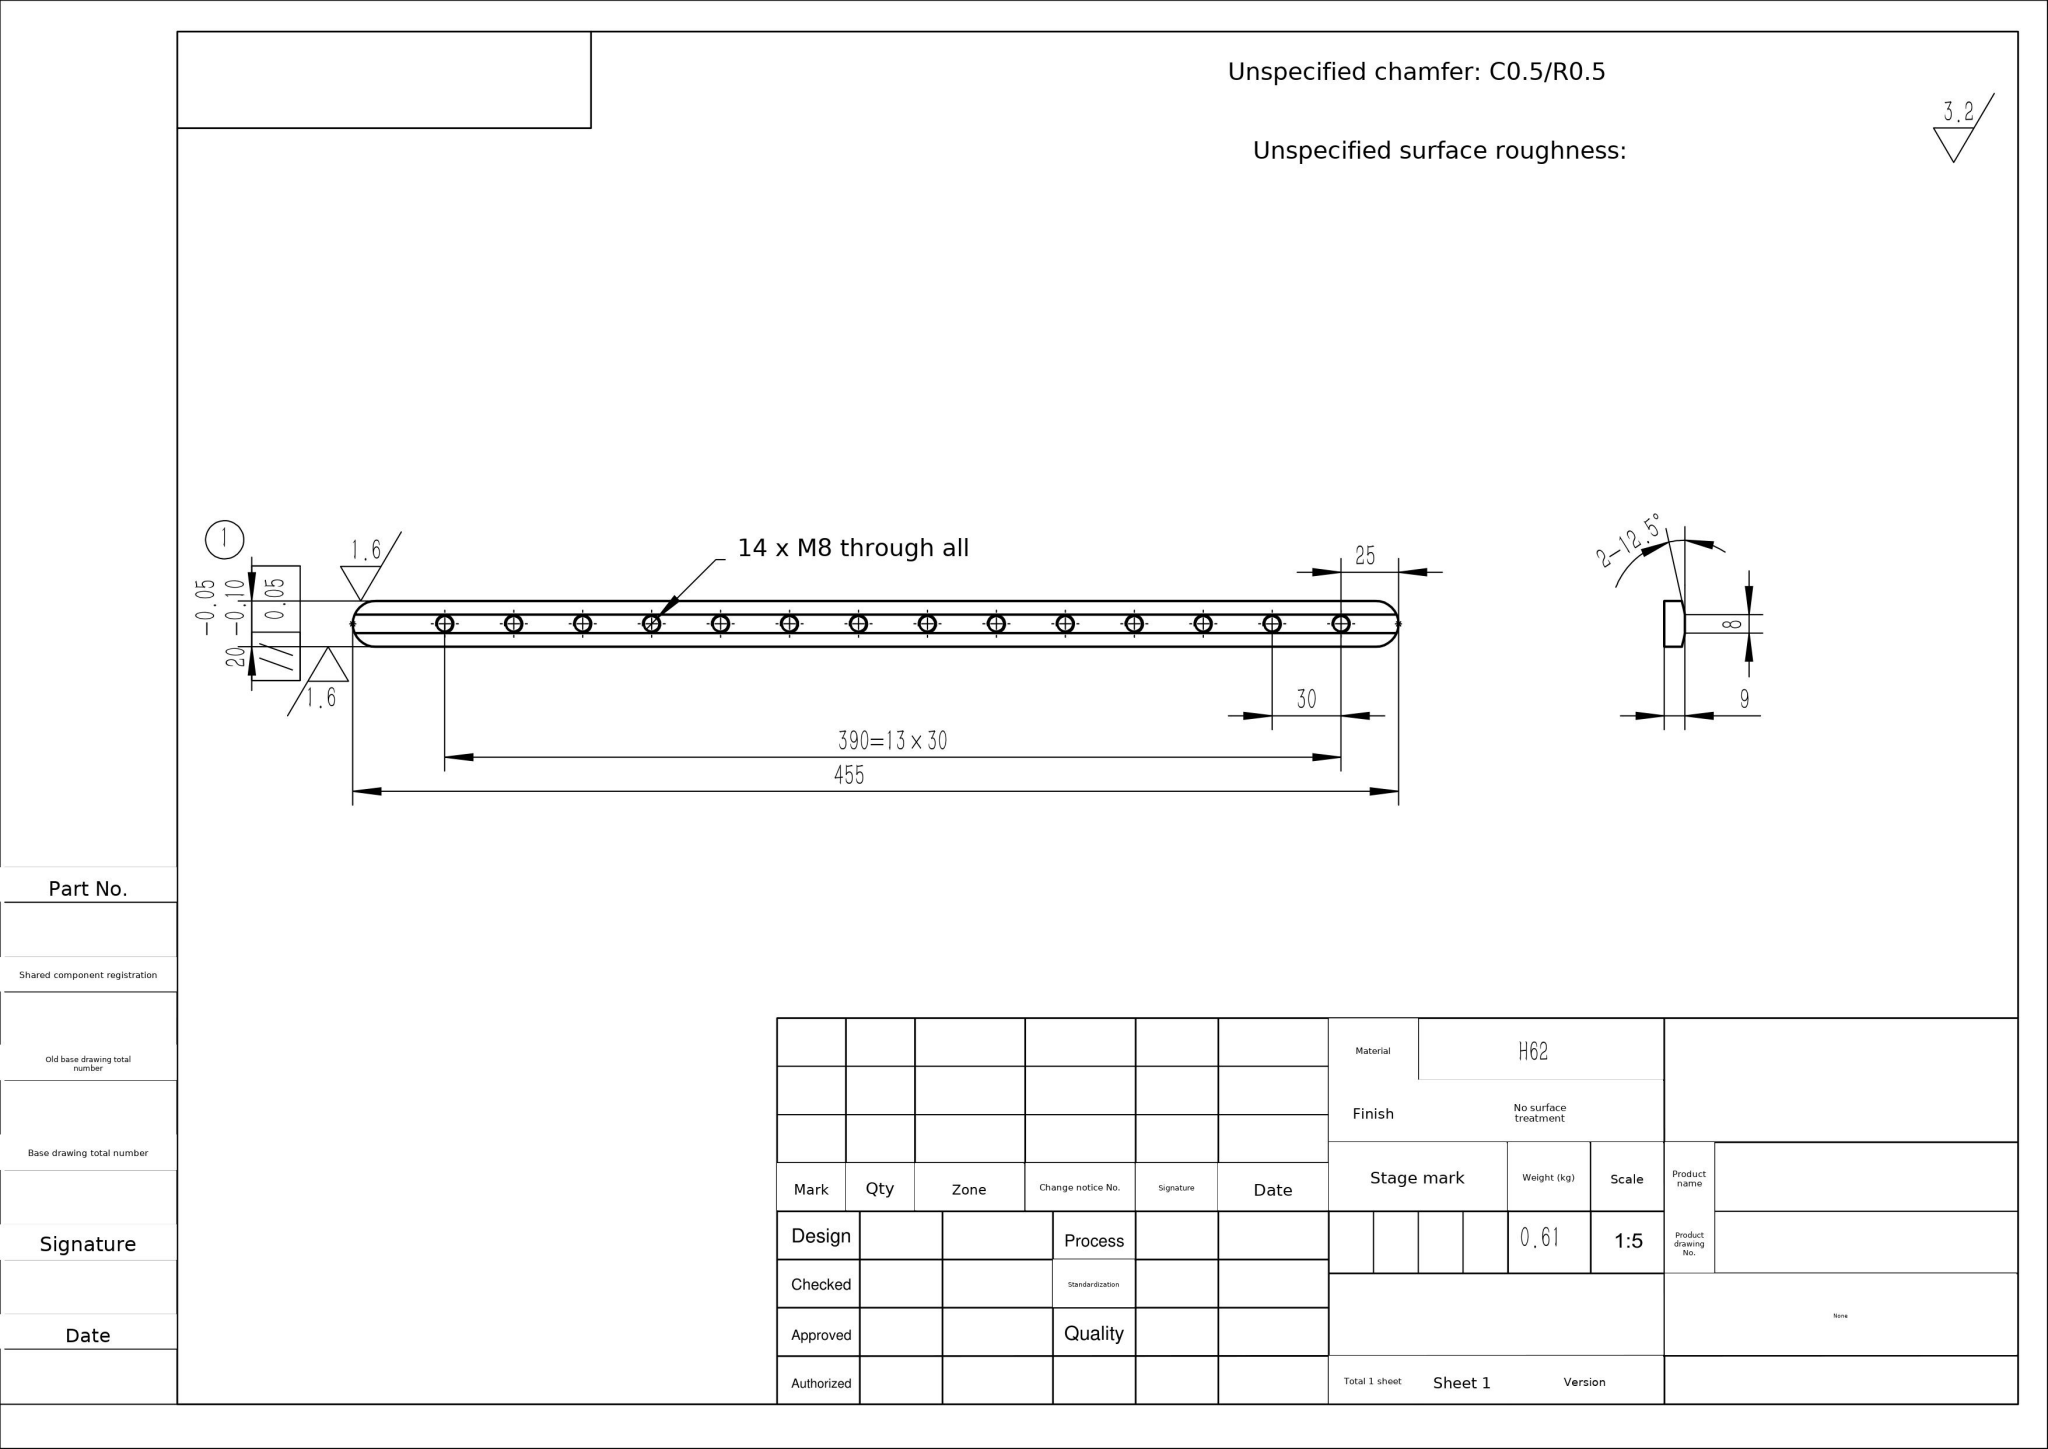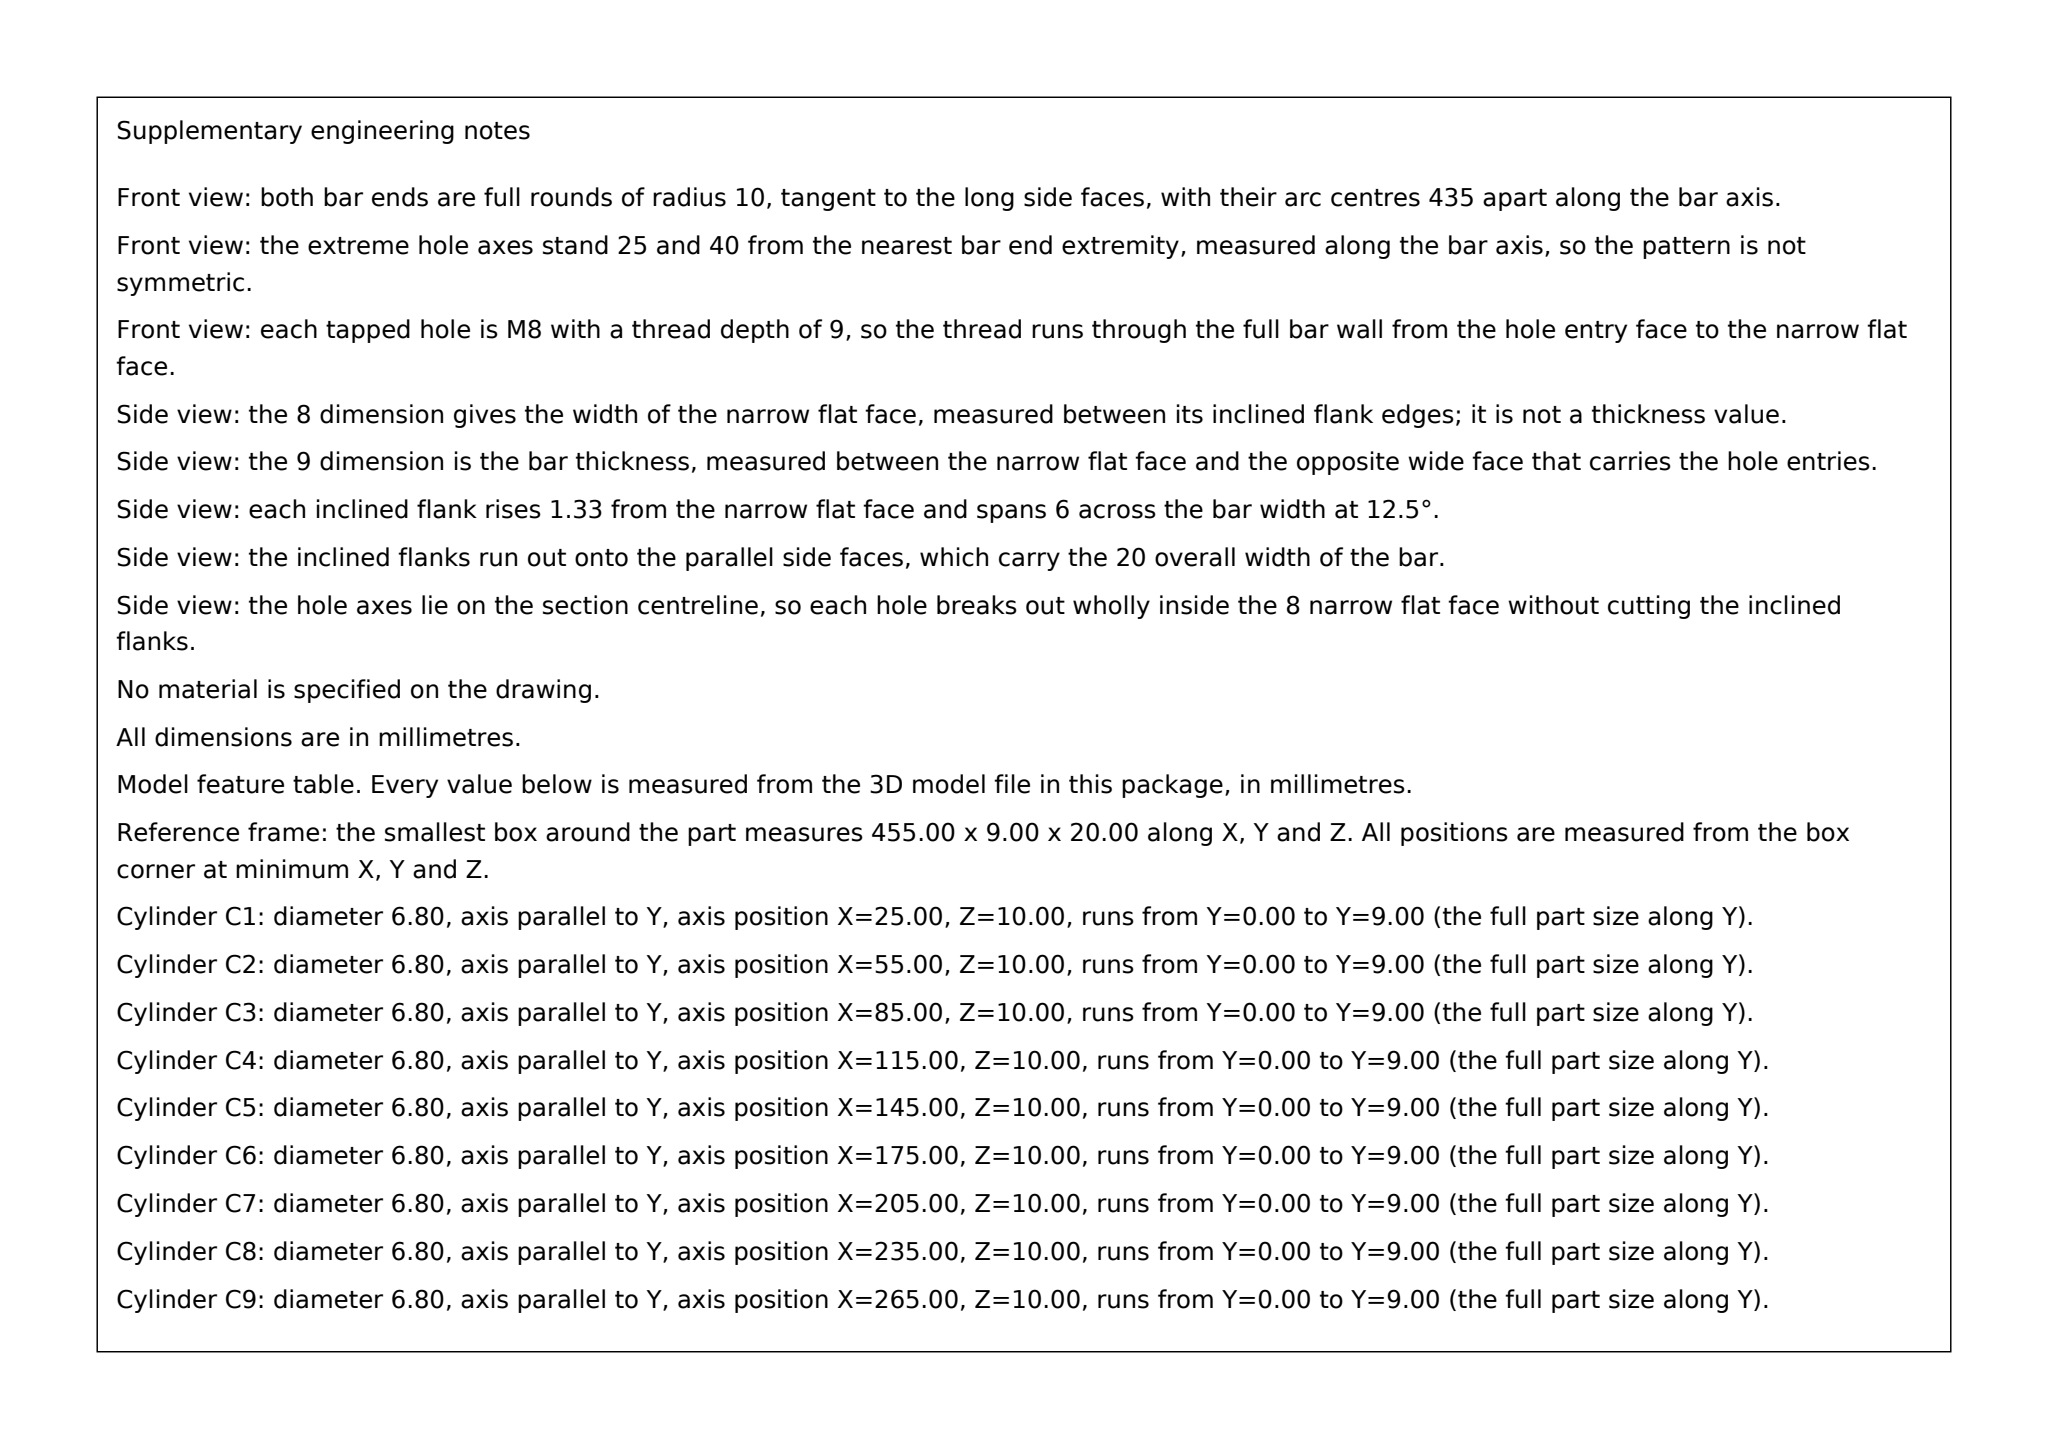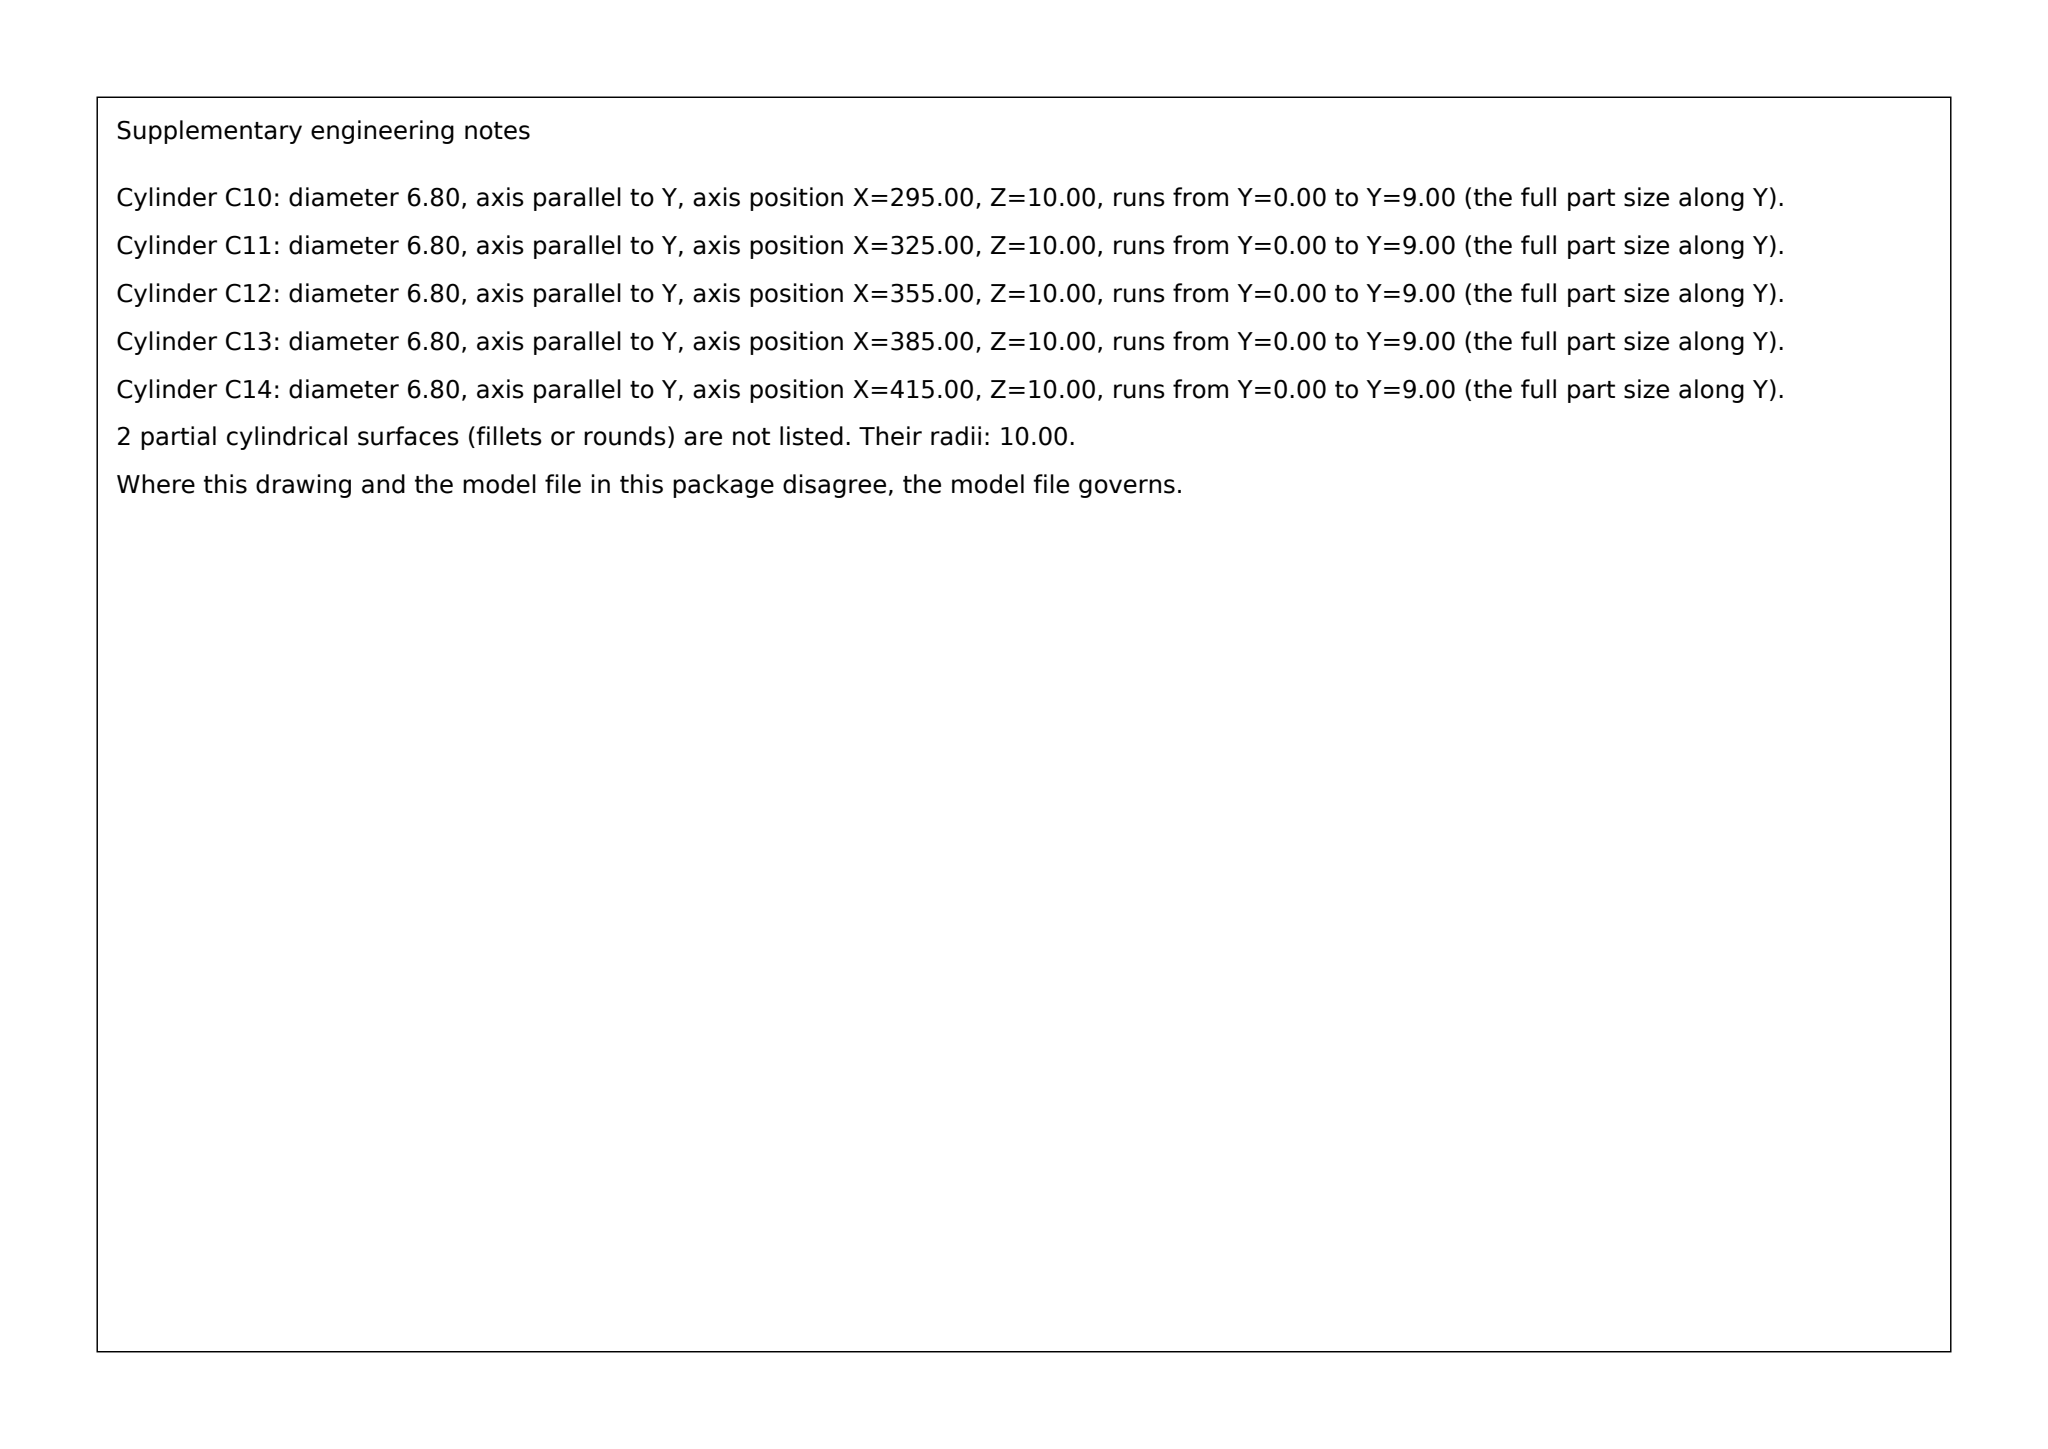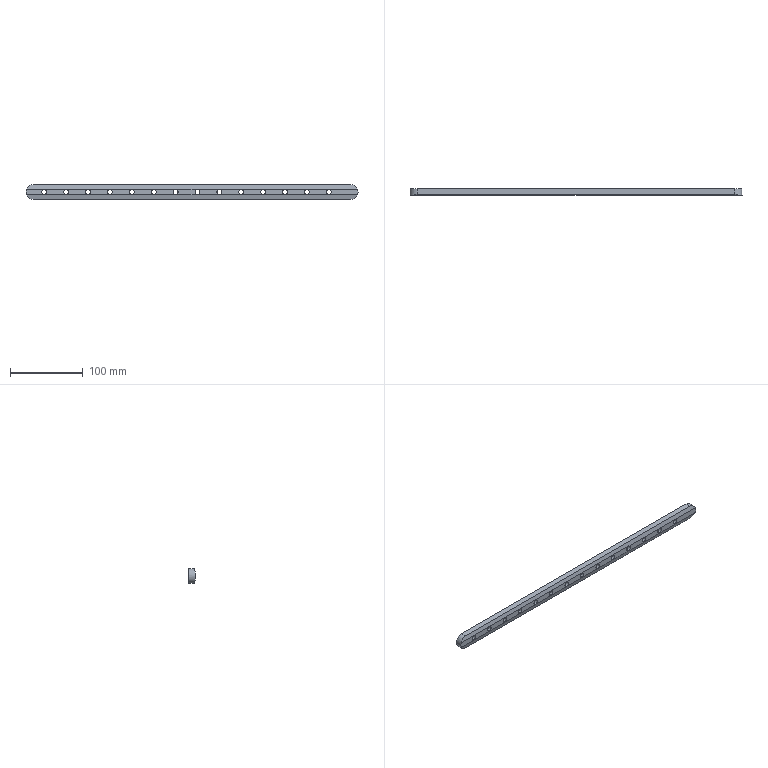Part | SolidWorks | mm | 1 solid | 36 faces | box 455 x 9 x 20 mm | volume 72993 mm3 | cylinder 30 | plane 6 | commonest cylinder face diameters 6.8 x28 20 x2
build123d program:
from build123d import *

# Parameters (mm, degrees)
BOSS_EXTRUDE1_DEPTH = 9
M8_TAPPED_HOLE1_D   = 6.8
LPATTERN1_COUNT     = 14
LPATTERN1_PITCH     = 30
CUT_EXTRUDE1_START  = -200
CUT_EXTRUDE1_DEPTH  = 555.279


with BuildPart() as part:
    # Sketch1 → Boss-Extrude1 (new body)
    with BuildSketch(Plane(origin=(0, 0, 0), x_dir=(1, 0, 0), z_dir=(0, 1, 0))):
        with BuildLine():
            Line((-90.977, 10), (344.023, 10))
            ThreePointArc((344.023, 10), (354.023, 0), (344.023, -10))
            Line((344.023, -10), (-90.977, -10))
            ThreePointArc((-90.977, -10), (-100.977, 0), (-90.977, 10))
        make_face()
    extrude(amount=BOSS_EXTRUDE1_DEPTH)

    # M8 Tapped Hole1 (through all)
    with Locations(Plane(origin=(0, 9, 0), x_dir=(1, 0, 0), z_dir=(0, 1, 0))):
        with Locations((-75.977, 0)):
            m8_tapped_hole1 = Hole(M8_TAPPED_HOLE1_D / 2)

    # LPattern1: M8 Tapped Hole1 ×14
    with Locations(*[(i * LPATTERN1_PITCH, 0, 0) for i in range(1, LPATTERN1_COUNT)]):
        add(m8_tapped_hole1, mode=Mode.SUBTRACT)

    # Sketch4 → Cut-Extrude1 (cut, through all)
    with BuildSketch(Plane(origin=(0, 0, 0), x_dir=(0, 0, -1), z_dir=(1, 0, 0)).offset(CUT_EXTRUDE1_START)):
        Polygon((4, 0), (14, 0), (14, 2.217), align=None)
        Polygon((-14, 2.217), (-14, 0), (-4, 0), align=None)
    extrude(amount=CUT_EXTRUDE1_DEPTH, mode=Mode.SUBTRACT)


solid = part.part